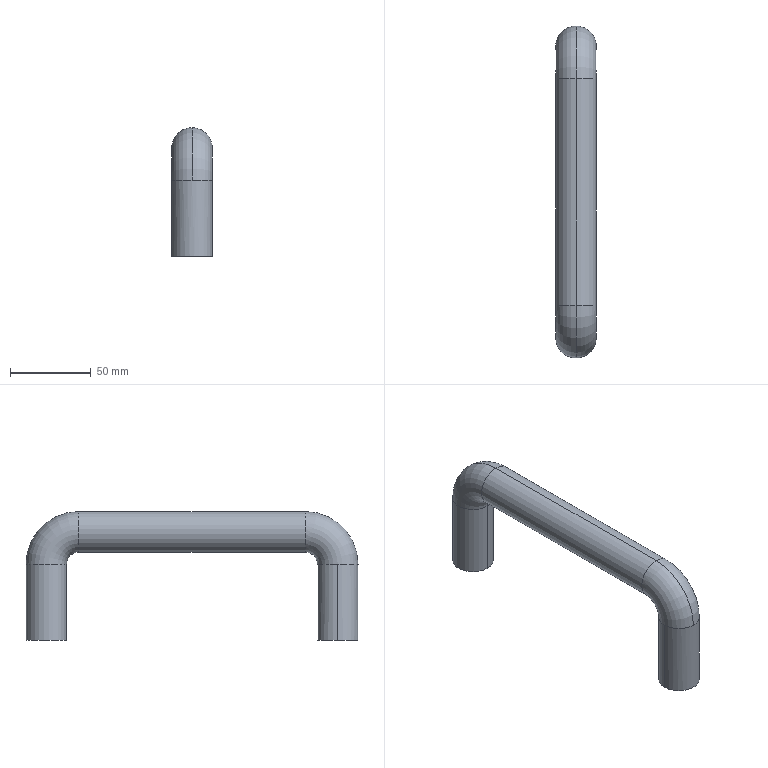Component | SolidWorks | Handle-1 | 1 solid | 18 faces | box 25 x 205 x 79.5 mm | volume 143162 mm3 | cylinder 10 | torus 4 | plane 4 | commonest cylinder face diameters 25 x6 9 x4
STEP:
#1=CARTESIAN_POINT('',(-13.762,-3.518,21.987));
#2=VERTEX_POINT('',#1);
#3=CARTESIAN_POINT('',(-13.762,-2.533,21.987));
#4=VERTEX_POINT('',#3);
#5=CARTESIAN_POINT('',(-13.762,-3.026,21.987));
#6=DIRECTION('',(0.,0.,1.));
#7=DIRECTION('',(1.,0.,0.));
#8=AXIS2_PLACEMENT_3D('',#5,#6,#7);
#9=CIRCLE('',#8,0.4921);
#10=EDGE_CURVE('',#2,#4,#9,.T.);
#11=ORIENTED_EDGE('',*,*,#10,.T.);
#12=CARTESIAN_POINT('',(-13.762,-3.813,23.267));
#13=VERTEX_POINT('',#12);
#14=CARTESIAN_POINT('',(-13.762,-3.813,21.987));
#15=DIRECTION('',(1.,0.,0.));
#16=DIRECTION('',(0.,0.,-1.));
#17=AXIS2_PLACEMENT_3D('',#14,#15,#16);
#18=CIRCLE('',#17,1.28);
#19=EDGE_CURVE('',#4,#13,#18,.T.);
#20=ORIENTED_EDGE('',*,*,#19,.T.);
#21=CARTESIAN_POINT('',(-13.762,-3.813,22.283));
#22=VERTEX_POINT('',#21);
#23=CARTESIAN_POINT('',(-13.762,-3.813,22.775));
#24=DIRECTION('',(0.,-1.,-0.));
#25=DIRECTION('',(1.,0.,0.));
#26=AXIS2_PLACEMENT_3D('',#23,#24,#25);
#27=CIRCLE('',#26,0.4921);
#28=EDGE_CURVE('',#22,#13,#27,.T.);
#29=ORIENTED_EDGE('',*,*,#28,.F.);
#30=CARTESIAN_POINT('',(-13.762,-3.813,21.987));
#31=DIRECTION('',(1.,0.,0.));
#32=DIRECTION('',(0.,0.,-1.));
#33=AXIS2_PLACEMENT_3D('',#30,#31,#32);
#34=CIRCLE('',#33,0.2953);
#35=EDGE_CURVE('',#2,#22,#34,.T.);
#36=ORIENTED_EDGE('',*,*,#35,.F.);
#37=EDGE_LOOP('',(#11,#20,#29,#36));
#38=FACE_OUTER_BOUND('',#37,.T.);
#39=CARTESIAN_POINT('',(-13.762,-3.813,21.987));
#40=DIRECTION('',(1.,0.,0.));
#41=DIRECTION('',(0.,0.,-1.));
#42=AXIS2_PLACEMENT_3D('',#39,#40,#41);
#43=TOROIDAL_SURFACE('',#42,0.7874,0.4921);
#44=ADVANCED_FACE('',(#38),#43,.T.);
#45=CARTESIAN_POINT('',(-13.762,-9.325,22.283));
#46=VERTEX_POINT('',#45);
#47=CARTESIAN_POINT('',(-13.762,-9.325,23.267));
#48=VERTEX_POINT('',#47);
#49=CARTESIAN_POINT('',(-13.762,-9.325,22.775));
#50=DIRECTION('',(0.,-1.,-0.));
#51=DIRECTION('',(1.,0.,0.));
#52=AXIS2_PLACEMENT_3D('',#49,#50,#51);
#53=CIRCLE('',#52,0.4921);
#54=EDGE_CURVE('',#46,#48,#53,.T.);
#55=ORIENTED_EDGE('',*,*,#54,.T.);
#56=CARTESIAN_POINT('',(-13.762,-10.604,21.987));
#57=VERTEX_POINT('',#56);
#58=CARTESIAN_POINT('',(-13.762,-9.325,21.987));
#59=DIRECTION('',(1.,0.,0.));
#60=DIRECTION('',(0.,0.,-1.));
#61=AXIS2_PLACEMENT_3D('',#58,#59,#60);
#62=CIRCLE('',#61,1.28);
#63=EDGE_CURVE('',#48,#57,#62,.T.);
#64=ORIENTED_EDGE('',*,*,#63,.T.);
#65=CARTESIAN_POINT('',(-13.27,-10.112,21.987));
#66=VERTEX_POINT('',#65);
#67=CARTESIAN_POINT('',(-13.762,-10.112,21.987));
#68=DIRECTION('',(0.,-0.,-1.));
#69=DIRECTION('',(1.,0.,0.));
#70=AXIS2_PLACEMENT_3D('',#67,#68,#69);
#71=CIRCLE('',#70,0.4921);
#72=EDGE_CURVE('',#66,#57,#71,.T.);
#73=ORIENTED_EDGE('',*,*,#72,.F.);
#74=CARTESIAN_POINT('',(-13.762,-9.62,21.987));
#75=VERTEX_POINT('',#74);
#76=CARTESIAN_POINT('',(-13.762,-10.112,21.987));
#77=DIRECTION('',(0.,-0.,-1.));
#78=DIRECTION('',(1.,0.,0.));
#79=AXIS2_PLACEMENT_3D('',#76,#77,#78);
#80=CIRCLE('',#79,0.4921);
#81=EDGE_CURVE('',#75,#66,#80,.T.);
#82=ORIENTED_EDGE('',*,*,#81,.F.);
#83=CARTESIAN_POINT('',(-13.762,-9.325,21.987));
#84=DIRECTION('',(1.,0.,0.));
#85=DIRECTION('',(0.,0.,-1.));
#86=AXIS2_PLACEMENT_3D('',#83,#84,#85);
#87=CIRCLE('',#86,0.2953);
#88=EDGE_CURVE('',#46,#75,#87,.T.);
#89=ORIENTED_EDGE('',*,*,#88,.F.);
#90=EDGE_LOOP('',(#55,#64,#73,#82,#89));
#91=FACE_OUTER_BOUND('',#90,.T.);
#92=CARTESIAN_POINT('',(-13.762,-9.325,21.987));
#93=DIRECTION('',(1.,0.,0.));
#94=DIRECTION('',(0.,0.,-1.));
#95=AXIS2_PLACEMENT_3D('',#92,#93,#94);
#96=TOROIDAL_SURFACE('',#95,0.7874,0.4921);
#97=ADVANCED_FACE('',(#91),#96,.T.);
#98=CARTESIAN_POINT('',(-13.585,-10.112,20.924));
#99=VERTEX_POINT('',#98);
#100=CARTESIAN_POINT('',(-13.939,-10.112,20.924));
#101=VERTEX_POINT('',#100);
#102=CARTESIAN_POINT('',(-13.762,-10.112,20.924));
#103=DIRECTION('',(0.,0.,-1.));
#104=DIRECTION('',(-1.,0.,0.));
#105=AXIS2_PLACEMENT_3D('',#102,#103,#104);
#106=CIRCLE('',#105,0.1772);
#107=EDGE_CURVE('',#99,#101,#106,.T.);
#108=ORIENTED_EDGE('',*,*,#107,.F.);
#109=CARTESIAN_POINT('',(-13.585,-10.112,20.137));
#110=VERTEX_POINT('',#109);
#111=CARTESIAN_POINT('',(-13.585,-10.112,20.924));
#112=DIRECTION('',(0.,0.,-1.));
#113=VECTOR('',#112,39.37);
#114=LINE('',#111,#113);
#115=EDGE_CURVE('',#99,#110,#114,.T.);
#116=ORIENTED_EDGE('',*,*,#115,.T.);
#117=CARTESIAN_POINT('',(-13.939,-10.112,20.137));
#118=VERTEX_POINT('',#117);
#119=CARTESIAN_POINT('',(-13.762,-10.112,20.137));
#120=DIRECTION('',(0.,0.,-1.));
#121=DIRECTION('',(-1.,0.,0.));
#122=AXIS2_PLACEMENT_3D('',#119,#120,#121);
#123=CIRCLE('',#122,0.1772);
#124=EDGE_CURVE('',#110,#118,#123,.T.);
#125=ORIENTED_EDGE('',*,*,#124,.T.);
#126=CARTESIAN_POINT('',(-13.939,-10.112,20.924));
#127=DIRECTION('',(0.,0.,-1.));
#128=VECTOR('',#127,39.37);
#129=LINE('',#126,#128);
#130=EDGE_CURVE('',#101,#118,#129,.T.);
#131=ORIENTED_EDGE('',*,*,#130,.F.);
#132=EDGE_LOOP('',(#108,#116,#125,#131));
#133=FACE_OUTER_BOUND('',#132,.T.);
#134=CARTESIAN_POINT('',(-13.762,-10.112,20.924));
#135=DIRECTION('',(0.,0.,-1.));
#136=DIRECTION('',(-1.,0.,0.));
#137=AXIS2_PLACEMENT_3D('',#134,#135,#136);
#138=CYLINDRICAL_SURFACE('',#137,0.1772);
#139=ADVANCED_FACE('',(#133),#138,.F.);
#140=CARTESIAN_POINT('',(-13.585,-3.026,20.924));
#141=VERTEX_POINT('',#140);
#142=CARTESIAN_POINT('',(-13.939,-3.026,20.924));
#143=VERTEX_POINT('',#142);
#144=CARTESIAN_POINT('',(-13.762,-3.026,20.924));
#145=DIRECTION('',(0.,0.,-1.));
#146=DIRECTION('',(-1.,0.,0.));
#147=AXIS2_PLACEMENT_3D('',#144,#145,#146);
#148=CIRCLE('',#147,0.1772);
#149=EDGE_CURVE('',#141,#143,#148,.T.);
#150=ORIENTED_EDGE('',*,*,#149,.F.);
#151=CARTESIAN_POINT('',(-13.585,-3.026,20.137));
#152=VERTEX_POINT('',#151);
#153=CARTESIAN_POINT('',(-13.585,-3.026,20.924));
#154=DIRECTION('',(0.,0.,-1.));
#155=VECTOR('',#154,39.37);
#156=LINE('',#153,#155);
#157=EDGE_CURVE('',#141,#152,#156,.T.);
#158=ORIENTED_EDGE('',*,*,#157,.T.);
#159=CARTESIAN_POINT('',(-13.939,-3.026,20.137));
#160=VERTEX_POINT('',#159);
#161=CARTESIAN_POINT('',(-13.762,-3.026,20.137));
#162=DIRECTION('',(0.,0.,-1.));
#163=DIRECTION('',(-1.,0.,0.));
#164=AXIS2_PLACEMENT_3D('',#161,#162,#163);
#165=CIRCLE('',#164,0.1772);
#166=EDGE_CURVE('',#152,#160,#165,.T.);
#167=ORIENTED_EDGE('',*,*,#166,.T.);
#168=CARTESIAN_POINT('',(-13.939,-3.026,20.924));
#169=DIRECTION('',(0.,0.,-1.));
#170=VECTOR('',#169,39.37);
#171=LINE('',#168,#170);
#172=EDGE_CURVE('',#143,#160,#171,.T.);
#173=ORIENTED_EDGE('',*,*,#172,.F.);
#174=EDGE_LOOP('',(#150,#158,#167,#173));
#175=FACE_OUTER_BOUND('',#174,.T.);
#176=CARTESIAN_POINT('',(-13.762,-3.026,20.924));
#177=DIRECTION('',(0.,0.,-1.));
#178=DIRECTION('',(-1.,0.,0.));
#179=AXIS2_PLACEMENT_3D('',#176,#177,#178);
#180=CYLINDRICAL_SURFACE('',#179,0.1772);
#181=ADVANCED_FACE('',(#175),#180,.F.);
#182=ORIENTED_EDGE('',*,*,#10,.F.);
#183=CARTESIAN_POINT('',(-13.762,-3.518,20.137));
#184=VERTEX_POINT('',#183);
#185=CARTESIAN_POINT('',(-13.762,-3.518,21.987));
#186=DIRECTION('',(0.,0.,-1.));
#187=VECTOR('',#186,39.37);
#188=LINE('',#185,#187);
#189=EDGE_CURVE('',#2,#184,#188,.T.);
#190=ORIENTED_EDGE('',*,*,#189,.T.);
#191=CARTESIAN_POINT('',(-13.762,-2.533,20.137));
#192=VERTEX_POINT('',#191);
#193=CARTESIAN_POINT('',(-13.762,-3.026,20.137));
#194=DIRECTION('',(0.,0.,1.));
#195=DIRECTION('',(1.,0.,0.));
#196=AXIS2_PLACEMENT_3D('',#193,#194,#195);
#197=CIRCLE('',#196,0.4921);
#198=EDGE_CURVE('',#184,#192,#197,.T.);
#199=ORIENTED_EDGE('',*,*,#198,.T.);
#200=CARTESIAN_POINT('',(-13.762,-2.533,21.987));
#201=DIRECTION('',(0.,0.,-1.));
#202=VECTOR('',#201,39.37);
#203=LINE('',#200,#202);
#204=EDGE_CURVE('',#4,#192,#203,.T.);
#205=ORIENTED_EDGE('',*,*,#204,.F.);
#206=EDGE_LOOP('',(#182,#190,#199,#205));
#207=FACE_OUTER_BOUND('',#206,.T.);
#208=CARTESIAN_POINT('',(-13.762,-3.026,21.987));
#209=DIRECTION('',(0.,0.,-1.));
#210=DIRECTION('',(0.,1.,0.));
#211=AXIS2_PLACEMENT_3D('',#208,#209,#210);
#212=CYLINDRICAL_SURFACE('',#211,0.4921);
#213=ADVANCED_FACE('',(#207),#212,.T.);
#214=ORIENTED_EDGE('',*,*,#28,.T.);
#215=CARTESIAN_POINT('',(-13.762,-3.813,23.267));
#216=DIRECTION('',(0.,-1.,-0.));
#217=VECTOR('',#216,39.37);
#218=LINE('',#215,#217);
#219=EDGE_CURVE('',#13,#48,#218,.T.);
#220=ORIENTED_EDGE('',*,*,#219,.T.);
#221=ORIENTED_EDGE('',*,*,#54,.F.);
#222=CARTESIAN_POINT('',(-13.762,-3.813,22.283));
#223=DIRECTION('',(0.,-1.,-0.));
#224=VECTOR('',#223,39.37);
#225=LINE('',#222,#224);
#226=EDGE_CURVE('',#22,#46,#225,.T.);
#227=ORIENTED_EDGE('',*,*,#226,.F.);
#228=EDGE_LOOP('',(#214,#220,#221,#227));
#229=FACE_OUTER_BOUND('',#228,.T.);
#230=CARTESIAN_POINT('',(-13.762,-3.813,22.775));
#231=DIRECTION('',(0.,-1.,-0.));
#232=DIRECTION('',(0.,0.,-1.));
#233=AXIS2_PLACEMENT_3D('',#230,#231,#232);
#234=CYLINDRICAL_SURFACE('',#233,0.4921);
#235=ADVANCED_FACE('',(#229),#234,.T.);
#236=CARTESIAN_POINT('',(-14.254,-10.112,21.987));
#237=VERTEX_POINT('',#236);
#238=CARTESIAN_POINT('',(-13.762,-10.112,21.987));
#239=DIRECTION('',(0.,-0.,-1.));
#240=DIRECTION('',(1.,0.,0.));
#241=AXIS2_PLACEMENT_3D('',#238,#239,#240);
#242=CIRCLE('',#241,0.4921);
#243=EDGE_CURVE('',#237,#75,#242,.T.);
#244=ORIENTED_EDGE('',*,*,#243,.T.);
#245=ORIENTED_EDGE('',*,*,#81,.T.);
#246=CARTESIAN_POINT('',(-13.27,-10.112,20.137));
#247=VERTEX_POINT('',#246);
#248=CARTESIAN_POINT('',(-13.27,-10.112,21.987));
#249=DIRECTION('',(0.,0.,-1.));
#250=VECTOR('',#249,39.37);
#251=LINE('',#248,#250);
#252=EDGE_CURVE('',#66,#247,#251,.T.);
#253=ORIENTED_EDGE('',*,*,#252,.T.);
#254=CARTESIAN_POINT('',(-14.254,-10.112,20.137));
#255=VERTEX_POINT('',#254);
#256=CARTESIAN_POINT('',(-13.762,-10.112,20.137));
#257=DIRECTION('',(0.,-0.,-1.));
#258=DIRECTION('',(1.,0.,0.));
#259=AXIS2_PLACEMENT_3D('',#256,#257,#258);
#260=CIRCLE('',#259,0.4921);
#261=EDGE_CURVE('',#255,#247,#260,.T.);
#262=ORIENTED_EDGE('',*,*,#261,.F.);
#263=CARTESIAN_POINT('',(-14.254,-10.112,21.987));
#264=DIRECTION('',(0.,0.,-1.));
#265=VECTOR('',#264,39.37);
#266=LINE('',#263,#265);
#267=EDGE_CURVE('',#237,#255,#266,.T.);
#268=ORIENTED_EDGE('',*,*,#267,.F.);
#269=EDGE_LOOP('',(#244,#245,#253,#262,#268));
#270=FACE_OUTER_BOUND('',#269,.T.);
#271=CARTESIAN_POINT('',(-13.762,-10.112,21.987));
#272=DIRECTION('',(0.,0.,-1.));
#273=DIRECTION('',(-1.,0.,0.));
#274=AXIS2_PLACEMENT_3D('',#271,#272,#273);
#275=CYLINDRICAL_SURFACE('',#274,0.4921);
#276=ADVANCED_FACE('',(#270),#275,.T.);
#277=ORIENTED_EDGE('',*,*,#252,.F.);
#278=ORIENTED_EDGE('',*,*,#72,.T.);
#279=CARTESIAN_POINT('',(-13.762,-10.112,21.987));
#280=DIRECTION('',(0.,-0.,-1.));
#281=DIRECTION('',(1.,0.,0.));
#282=AXIS2_PLACEMENT_3D('',#279,#280,#281);
#283=CIRCLE('',#282,0.4921);
#284=EDGE_CURVE('',#57,#237,#283,.T.);
#285=ORIENTED_EDGE('',*,*,#284,.T.);
#286=ORIENTED_EDGE('',*,*,#267,.T.);
#287=CARTESIAN_POINT('',(-13.762,-10.112,20.137));
#288=DIRECTION('',(0.,-0.,-1.));
#289=DIRECTION('',(1.,0.,0.));
#290=AXIS2_PLACEMENT_3D('',#287,#288,#289);
#291=CIRCLE('',#290,0.4921);
#292=EDGE_CURVE('',#247,#255,#291,.T.);
#293=ORIENTED_EDGE('',*,*,#292,.F.);
#294=EDGE_LOOP('',(#277,#278,#285,#286,#293));
#295=FACE_OUTER_BOUND('',#294,.T.);
#296=CARTESIAN_POINT('',(-13.762,-10.112,21.987));
#297=DIRECTION('',(0.,0.,-1.));
#298=DIRECTION('',(-1.,0.,0.));
#299=AXIS2_PLACEMENT_3D('',#296,#297,#298);
#300=CYLINDRICAL_SURFACE('',#299,0.4921);
#301=ADVANCED_FACE('',(#295),#300,.T.);
#302=ORIENTED_EDGE('',*,*,#63,.F.);
#303=CARTESIAN_POINT('',(-13.762,-9.325,22.775));
#304=DIRECTION('',(0.,-1.,-0.));
#305=DIRECTION('',(1.,0.,0.));
#306=AXIS2_PLACEMENT_3D('',#303,#304,#305);
#307=CIRCLE('',#306,0.4921);
#308=EDGE_CURVE('',#48,#46,#307,.T.);
#309=ORIENTED_EDGE('',*,*,#308,.T.);
#310=ORIENTED_EDGE('',*,*,#88,.T.);
#311=ORIENTED_EDGE('',*,*,#243,.F.);
#312=ORIENTED_EDGE('',*,*,#284,.F.);
#313=EDGE_LOOP('',(#302,#309,#310,#311,#312));
#314=FACE_OUTER_BOUND('',#313,.T.);
#315=CARTESIAN_POINT('',(-13.762,-9.325,21.987));
#316=DIRECTION('',(1.,0.,0.));
#317=DIRECTION('',(0.,0.,-1.));
#318=AXIS2_PLACEMENT_3D('',#315,#316,#317);
#319=TOROIDAL_SURFACE('',#318,0.7874,0.4921);
#320=ADVANCED_FACE('',(#314),#319,.T.);
#321=ORIENTED_EDGE('',*,*,#219,.F.);
#322=CARTESIAN_POINT('',(-13.762,-3.813,22.775));
#323=DIRECTION('',(0.,-1.,-0.));
#324=DIRECTION('',(1.,0.,0.));
#325=AXIS2_PLACEMENT_3D('',#322,#323,#324);
#326=CIRCLE('',#325,0.4921);
#327=EDGE_CURVE('',#13,#22,#326,.T.);
#328=ORIENTED_EDGE('',*,*,#327,.T.);
#329=ORIENTED_EDGE('',*,*,#226,.T.);
#330=ORIENTED_EDGE('',*,*,#308,.F.);
#331=EDGE_LOOP('',(#321,#328,#329,#330));
#332=FACE_OUTER_BOUND('',#331,.T.);
#333=CARTESIAN_POINT('',(-13.762,-3.813,22.775));
#334=DIRECTION('',(0.,-1.,-0.));
#335=DIRECTION('',(0.,0.,-1.));
#336=AXIS2_PLACEMENT_3D('',#333,#334,#335);
#337=CYLINDRICAL_SURFACE('',#336,0.4921);
#338=ADVANCED_FACE('',(#332),#337,.T.);
#339=ORIENTED_EDGE('',*,*,#19,.F.);
#340=CARTESIAN_POINT('',(-13.762,-3.026,21.987));
#341=DIRECTION('',(0.,0.,1.));
#342=DIRECTION('',(1.,0.,0.));
#343=AXIS2_PLACEMENT_3D('',#340,#341,#342);
#344=CIRCLE('',#343,0.4921);
#345=EDGE_CURVE('',#4,#2,#344,.T.);
#346=ORIENTED_EDGE('',*,*,#345,.T.);
#347=ORIENTED_EDGE('',*,*,#35,.T.);
#348=ORIENTED_EDGE('',*,*,#327,.F.);
#349=EDGE_LOOP('',(#339,#346,#347,#348));
#350=FACE_OUTER_BOUND('',#349,.T.);
#351=CARTESIAN_POINT('',(-13.762,-3.813,21.987));
#352=DIRECTION('',(1.,0.,0.));
#353=DIRECTION('',(0.,0.,-1.));
#354=AXIS2_PLACEMENT_3D('',#351,#352,#353);
#355=TOROIDAL_SURFACE('',#354,0.7874,0.4921);
#356=ADVANCED_FACE('',(#350),#355,.T.);
#357=ORIENTED_EDGE('',*,*,#189,.F.);
#358=ORIENTED_EDGE('',*,*,#345,.F.);
#359=ORIENTED_EDGE('',*,*,#204,.T.);
#360=CARTESIAN_POINT('',(-13.762,-3.026,20.137));
#361=DIRECTION('',(0.,0.,1.));
#362=DIRECTION('',(1.,0.,0.));
#363=AXIS2_PLACEMENT_3D('',#360,#361,#362);
#364=CIRCLE('',#363,0.4921);
#365=EDGE_CURVE('',#192,#184,#364,.T.);
#366=ORIENTED_EDGE('',*,*,#365,.T.);
#367=EDGE_LOOP('',(#357,#358,#359,#366));
#368=FACE_OUTER_BOUND('',#367,.T.);
#369=CARTESIAN_POINT('',(-13.762,-3.026,21.987));
#370=DIRECTION('',(0.,0.,-1.));
#371=DIRECTION('',(0.,1.,0.));
#372=AXIS2_PLACEMENT_3D('',#369,#370,#371);
#373=CYLINDRICAL_SURFACE('',#372,0.4921);
#374=ADVANCED_FACE('',(#368),#373,.T.);
#375=CARTESIAN_POINT('',(-13.762,-10.112,20.137));
#376=DIRECTION('',(0.,0.,-1.));
#377=DIRECTION('',(-1.,0.,0.));
#378=AXIS2_PLACEMENT_3D('',#375,#376,#377);
#379=CIRCLE('',#378,0.1772);
#380=EDGE_CURVE('',#118,#110,#379,.T.);
#381=ORIENTED_EDGE('',*,*,#380,.F.);
#382=ORIENTED_EDGE('',*,*,#124,.F.);
#383=EDGE_LOOP('',(#381,#382));
#384=FACE_BOUND('',#383,.T.);
#385=ORIENTED_EDGE('',*,*,#261,.T.);
#386=ORIENTED_EDGE('',*,*,#292,.T.);
#387=EDGE_LOOP('',(#385,#386));
#388=FACE_OUTER_BOUND('',#387,.T.);
#389=CARTESIAN_POINT('',(-13.762,-10.112,20.137));
#390=DIRECTION('',(0.,-0.,-1.));
#391=DIRECTION('',(1.,0.,0.));
#392=AXIS2_PLACEMENT_3D('',#389,#390,#391);
#393=PLANE('',#392);
#394=ADVANCED_FACE('',(#384,#388),#393,.T.);
#395=CARTESIAN_POINT('',(-13.762,-3.026,20.137));
#396=DIRECTION('',(0.,0.,-1.));
#397=DIRECTION('',(-1.,0.,0.));
#398=AXIS2_PLACEMENT_3D('',#395,#396,#397);
#399=CIRCLE('',#398,0.1772);
#400=EDGE_CURVE('',#160,#152,#399,.T.);
#401=ORIENTED_EDGE('',*,*,#400,.F.);
#402=ORIENTED_EDGE('',*,*,#166,.F.);
#403=EDGE_LOOP('',(#401,#402));
#404=FACE_BOUND('',#403,.T.);
#405=ORIENTED_EDGE('',*,*,#365,.F.);
#406=ORIENTED_EDGE('',*,*,#198,.F.);
#407=EDGE_LOOP('',(#405,#406));
#408=FACE_OUTER_BOUND('',#407,.T.);
#409=CARTESIAN_POINT('',(-13.762,-3.026,20.137));
#410=DIRECTION('',(0.,0.,1.));
#411=DIRECTION('',(1.,0.,0.));
#412=AXIS2_PLACEMENT_3D('',#409,#410,#411);
#413=PLANE('',#412);
#414=ADVANCED_FACE('',(#404,#408),#413,.F.);
#415=ORIENTED_EDGE('',*,*,#157,.F.);
#416=CARTESIAN_POINT('',(-13.762,-3.026,20.924));
#417=DIRECTION('',(0.,0.,-1.));
#418=DIRECTION('',(-1.,0.,0.));
#419=AXIS2_PLACEMENT_3D('',#416,#417,#418);
#420=CIRCLE('',#419,0.1772);
#421=EDGE_CURVE('',#143,#141,#420,.T.);
#422=ORIENTED_EDGE('',*,*,#421,.F.);
#423=ORIENTED_EDGE('',*,*,#172,.T.);
#424=ORIENTED_EDGE('',*,*,#400,.T.);
#425=EDGE_LOOP('',(#415,#422,#423,#424));
#426=FACE_OUTER_BOUND('',#425,.T.);
#427=CARTESIAN_POINT('',(-13.762,-3.026,20.924));
#428=DIRECTION('',(0.,0.,-1.));
#429=DIRECTION('',(-1.,0.,0.));
#430=AXIS2_PLACEMENT_3D('',#427,#428,#429);
#431=CYLINDRICAL_SURFACE('',#430,0.1772);
#432=ADVANCED_FACE('',(#426),#431,.F.);
#433=ORIENTED_EDGE('',*,*,#421,.T.);
#434=ORIENTED_EDGE('',*,*,#149,.T.);
#435=EDGE_LOOP('',(#433,#434));
#436=FACE_OUTER_BOUND('',#435,.T.);
#437=CARTESIAN_POINT('',(-13.762,-3.026,20.924));
#438=DIRECTION('',(0.,0.,-1.));
#439=DIRECTION('',(-1.,0.,0.));
#440=AXIS2_PLACEMENT_3D('',#437,#438,#439);
#441=PLANE('',#440);
#442=ADVANCED_FACE('',(#436),#441,.T.);
#443=ORIENTED_EDGE('',*,*,#115,.F.);
#444=CARTESIAN_POINT('',(-13.762,-10.112,20.924));
#445=DIRECTION('',(0.,0.,-1.));
#446=DIRECTION('',(-1.,0.,0.));
#447=AXIS2_PLACEMENT_3D('',#444,#445,#446);
#448=CIRCLE('',#447,0.1772);
#449=EDGE_CURVE('',#101,#99,#448,.T.);
#450=ORIENTED_EDGE('',*,*,#449,.F.);
#451=ORIENTED_EDGE('',*,*,#130,.T.);
#452=ORIENTED_EDGE('',*,*,#380,.T.);
#453=EDGE_LOOP('',(#443,#450,#451,#452));
#454=FACE_OUTER_BOUND('',#453,.T.);
#455=CARTESIAN_POINT('',(-13.762,-10.112,20.924));
#456=DIRECTION('',(0.,0.,-1.));
#457=DIRECTION('',(-1.,0.,0.));
#458=AXIS2_PLACEMENT_3D('',#455,#456,#457);
#459=CYLINDRICAL_SURFACE('',#458,0.1772);
#460=ADVANCED_FACE('',(#454),#459,.F.);
#461=ORIENTED_EDGE('',*,*,#449,.T.);
#462=ORIENTED_EDGE('',*,*,#107,.T.);
#463=EDGE_LOOP('',(#461,#462));
#464=FACE_OUTER_BOUND('',#463,.T.);
#465=CARTESIAN_POINT('',(-13.762,-10.112,20.924));
#466=DIRECTION('',(0.,0.,-1.));
#467=DIRECTION('',(-1.,0.,0.));
#468=AXIS2_PLACEMENT_3D('',#465,#466,#467);
#469=PLANE('',#468);
#470=ADVANCED_FACE('',(#464),#469,.T.);
#471=CLOSED_SHELL('',(#44,#97,#139,#181,#213,#235,#276,#301,#320,#338,#356,#374,#394,#414,#432,#442,#460,#470));
#472=MANIFOLD_SOLID_BREP('',#471);
#473=CARTESIAN_POINT('',(0.,0.,0.));
#474=DIRECTION('',(0.,0.,1.));
#475=DIRECTION('',(1.,0.,0.));
#476=AXIS2_PLACEMENT_3D('',#473,#474,#475);
#477=(LENGTH_UNIT()NAMED_UNIT(*)SI_UNIT($,.METRE.));
#478=LENGTH_MEASURE_WITH_UNIT(LENGTH_MEASURE(0.0254),#477);
#479=DIMENSIONAL_EXPONENTS(1.,0.,0.,0.,0.,0.,0.);
#480=(CONVERSION_BASED_UNIT('',#478)LENGTH_UNIT()NAMED_UNIT(#479));
#481=UNCERTAINTY_MEASURE_WITH_UNIT(LENGTH_MEASURE(0.00001),#480,'','');
#482=(NAMED_UNIT(*)PLANE_ANGLE_UNIT()SI_UNIT($,.RADIAN.));
#483=(NAMED_UNIT(*)SI_UNIT($,.STERADIAN.)SOLID_ANGLE_UNIT());
#484=(GEOMETRIC_REPRESENTATION_CONTEXT(3)GLOBAL_UNCERTAINTY_ASSIGNED_CONTEXT((#481))GLOBAL_UNIT_ASSIGNED_CONTEXT((#480,#482,#483))REPRESENTATION_CONTEXT('',''));
#485=ADVANCED_BREP_SHAPE_REPRESENTATION('',(#472,#476),#484);
#486=COLOUR_RGB('',0.7922,0.8196,0.9333);
#487=FILL_AREA_STYLE_COLOUR('',#486);
#488=FILL_AREA_STYLE('',(#487));
#489=SURFACE_STYLE_FILL_AREA(#488);
#490=SURFACE_SIDE_STYLE('',(#489));
#491=SURFACE_STYLE_USAGE(.BOTH.,#490);
#492=PRESENTATION_STYLE_ASSIGNMENT((#491));
#493=STYLED_ITEM('',(#492),#472);
#494=PRESENTATION_LAYER_ASSIGNMENT('','',(#493));
#495=(LENGTH_UNIT()NAMED_UNIT(*)SI_UNIT($,.METRE.));
#496=LENGTH_MEASURE_WITH_UNIT(LENGTH_MEASURE(0.0254),#495);
#497=DIMENSIONAL_EXPONENTS(1.,0.,0.,0.,0.,0.,0.);
#498=(CONVERSION_BASED_UNIT('',#496)LENGTH_UNIT()NAMED_UNIT(#497));
#499=UNCERTAINTY_MEASURE_WITH_UNIT(LENGTH_MEASURE(0.00001),#498,'','');
#500=(NAMED_UNIT(*)PLANE_ANGLE_UNIT()SI_UNIT($,.RADIAN.));
#501=(NAMED_UNIT(*)SI_UNIT($,.STERADIAN.)SOLID_ANGLE_UNIT());
#502=(GEOMETRIC_REPRESENTATION_CONTEXT(3)GLOBAL_UNCERTAINTY_ASSIGNED_CONTEXT((#499))GLOBAL_UNIT_ASSIGNED_CONTEXT((#498,#500,#501))REPRESENTATION_CONTEXT('',''));
#503=MECHANICAL_DESIGN_GEOMETRIC_PRESENTATION_REPRESENTATION('',(#493),#502);